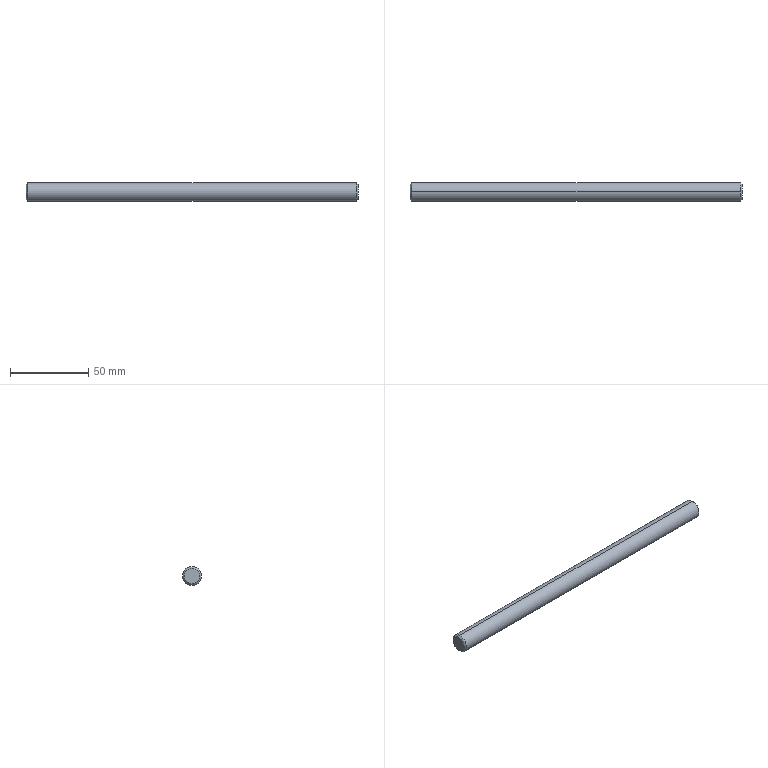Component | SolidWorks | PhotoelectricSlideRod-1 | 1 solid | 8 faces | box 212 x 12 x 12 mm | volume 23941 mm3 | cone 4 | cylinder 2 | plane 2 | commonest cylinder face diameters 12 x2
build123d program:
from build123d import *


with BuildPart() as part:
    # Sketch1 → Revolve1 (revolve)
    with BuildSketch(Plane(origin=(0, 0, 0), x_dir=(1, 0, 0), z_dir=(0, 1, 0))):
        Polygon((5, 106), (0, 106), (0, -106), (5, -106), (6, -105), (6, 105), align=None)
    revolve(axis=Axis((0, 0, -106), (0, 0, 1)))


solid = part.part

# Placed as in the assembly
solid = solid.moved(Location((170, 556, -227.5), (0, 90, 0)))
STEP:
#1=COLOUR_RGB('',0.7922,0.8196,0.9333);
#2=FILL_AREA_STYLE_COLOUR('',#1);
#3=FILL_AREA_STYLE('',(#2));
#4=SURFACE_STYLE_FILL_AREA(#3);
#5=SURFACE_SIDE_STYLE('',(#4));
#6=SURFACE_STYLE_USAGE(.BOTH.,#5);
#7=PRESENTATION_STYLE_ASSIGNMENT((#6));
#8=CARTESIAN_POINT('',(10.866,21.89,-9.154));
#9=VERTEX_POINT('',#8);
#10=CARTESIAN_POINT('',(10.866,21.89,-8.76));
#11=VERTEX_POINT('',#10);
#12=CARTESIAN_POINT('',(10.866,21.89,-8.957));
#13=DIRECTION('',(1.,0.,0.));
#14=DIRECTION('',(0.,0.,-1.));
#15=AXIS2_PLACEMENT_3D('',#12,#13,#14);
#16=CIRCLE('',#15,0.1969);
#17=EDGE_CURVE('',#9,#11,#16,.T.);
#18=ORIENTED_EDGE('',*,*,#17,.F.);
#19=CARTESIAN_POINT('',(10.827,21.89,-9.193));
#20=VERTEX_POINT('',#19);
#21=CARTESIAN_POINT('',(10.866,21.89,-9.154));
#22=DIRECTION('',(-0.7071,-0.,-0.7071));
#23=VECTOR('',#22,39.37);
#24=LINE('',#21,#23);
#25=EDGE_CURVE('',#9,#20,#24,.T.);
#26=ORIENTED_EDGE('',*,*,#25,.T.);
#27=CARTESIAN_POINT('',(10.827,21.89,-8.72));
#28=VERTEX_POINT('',#27);
#29=CARTESIAN_POINT('',(10.827,21.89,-8.957));
#30=DIRECTION('',(1.,0.,0.));
#31=DIRECTION('',(0.,0.,-1.));
#32=AXIS2_PLACEMENT_3D('',#29,#30,#31);
#33=CIRCLE('',#32,0.2362);
#34=EDGE_CURVE('',#20,#28,#33,.T.);
#35=ORIENTED_EDGE('',*,*,#34,.T.);
#36=CARTESIAN_POINT('',(10.866,21.89,-8.76));
#37=DIRECTION('',(-0.7071,-0.,0.7071));
#38=VECTOR('',#37,39.37);
#39=LINE('',#36,#38);
#40=EDGE_CURVE('',#11,#28,#39,.T.);
#41=ORIENTED_EDGE('',*,*,#40,.F.);
#42=EDGE_LOOP('',(#18,#26,#35,#41));
#43=FACE_OUTER_BOUND('',#42,.T.);
#44=CARTESIAN_POINT('',(10.866,21.89,-8.957));
#45=DIRECTION('',(-1.,-0.,0.));
#46=DIRECTION('',(0.,0.,1.));
#47=AXIS2_PLACEMENT_3D('',#44,#45,#46);
#48=CONICAL_SURFACE('',#47,0.1969,0.7854);
#49=ADVANCED_FACE('',(#43),#48,.T.);
#50=CARTESIAN_POINT('',(2.559,21.89,-9.193));
#51=VERTEX_POINT('',#50);
#52=CARTESIAN_POINT('',(2.559,21.89,-8.72));
#53=VERTEX_POINT('',#52);
#54=CARTESIAN_POINT('',(2.559,21.89,-8.957));
#55=DIRECTION('',(1.,0.,0.));
#56=DIRECTION('',(0.,0.,-1.));
#57=AXIS2_PLACEMENT_3D('',#54,#55,#56);
#58=CIRCLE('',#57,0.2362);
#59=EDGE_CURVE('',#51,#53,#58,.T.);
#60=ORIENTED_EDGE('',*,*,#59,.T.);
#61=CARTESIAN_POINT('',(2.52,21.89,-8.72));
#62=DIRECTION('',(1.,0.,0.));
#63=VECTOR('',#62,39.37);
#64=LINE('',#61,#63);
#65=EDGE_CURVE('',#53,#28,#64,.T.);
#66=ORIENTED_EDGE('',*,*,#65,.T.);
#67=ORIENTED_EDGE('',*,*,#34,.F.);
#68=CARTESIAN_POINT('',(2.52,21.89,-9.193));
#69=DIRECTION('',(1.,0.,0.));
#70=VECTOR('',#69,39.37);
#71=LINE('',#68,#70);
#72=EDGE_CURVE('',#51,#20,#71,.T.);
#73=ORIENTED_EDGE('',*,*,#72,.F.);
#74=EDGE_LOOP('',(#60,#66,#67,#73));
#75=FACE_OUTER_BOUND('',#74,.T.);
#76=CARTESIAN_POINT('',(2.52,21.89,-8.957));
#77=DIRECTION('',(1.,0.,0.));
#78=DIRECTION('',(0.,0.,-1.));
#79=AXIS2_PLACEMENT_3D('',#76,#77,#78);
#80=CYLINDRICAL_SURFACE('',#79,0.2362);
#81=ADVANCED_FACE('',(#75),#80,.T.);
#82=CARTESIAN_POINT('',(2.52,21.89,-9.154));
#83=VERTEX_POINT('',#82);
#84=CARTESIAN_POINT('',(2.52,21.89,-8.76));
#85=VERTEX_POINT('',#84);
#86=CARTESIAN_POINT('',(2.52,21.89,-8.957));
#87=DIRECTION('',(1.,0.,0.));
#88=DIRECTION('',(0.,0.,-1.));
#89=AXIS2_PLACEMENT_3D('',#86,#87,#88);
#90=CIRCLE('',#89,0.1969);
#91=EDGE_CURVE('',#83,#85,#90,.T.);
#92=ORIENTED_EDGE('',*,*,#91,.T.);
#93=CARTESIAN_POINT('',(2.559,21.89,-8.72));
#94=DIRECTION('',(0.7071,0.,0.7071));
#95=VECTOR('',#94,39.37);
#96=LINE('',#93,#95);
#97=EDGE_CURVE('',#85,#53,#96,.T.);
#98=ORIENTED_EDGE('',*,*,#97,.T.);
#99=ORIENTED_EDGE('',*,*,#59,.F.);
#100=CARTESIAN_POINT('',(2.559,21.89,-9.193));
#101=DIRECTION('',(0.7071,-0.,-0.7071));
#102=VECTOR('',#101,39.37);
#103=LINE('',#100,#102);
#104=EDGE_CURVE('',#83,#51,#103,.T.);
#105=ORIENTED_EDGE('',*,*,#104,.F.);
#106=EDGE_LOOP('',(#92,#98,#99,#105));
#107=FACE_OUTER_BOUND('',#106,.T.);
#108=CARTESIAN_POINT('',(2.559,21.89,-8.957));
#109=DIRECTION('',(1.,0.,0.));
#110=DIRECTION('',(0.,0.,-1.));
#111=AXIS2_PLACEMENT_3D('',#108,#109,#110);
#112=CONICAL_SURFACE('',#111,0.2362,0.7854);
#113=ADVANCED_FACE('',(#107),#112,.T.);
#114=ORIENTED_EDGE('',*,*,#97,.F.);
#115=CARTESIAN_POINT('',(2.52,21.89,-8.957));
#116=DIRECTION('',(1.,0.,0.));
#117=DIRECTION('',(0.,0.,-1.));
#118=AXIS2_PLACEMENT_3D('',#115,#116,#117);
#119=CIRCLE('',#118,0.1969);
#120=EDGE_CURVE('',#85,#83,#119,.T.);
#121=ORIENTED_EDGE('',*,*,#120,.T.);
#122=ORIENTED_EDGE('',*,*,#104,.T.);
#123=CARTESIAN_POINT('',(2.559,21.89,-8.957));
#124=DIRECTION('',(1.,0.,0.));
#125=DIRECTION('',(0.,0.,-1.));
#126=AXIS2_PLACEMENT_3D('',#123,#124,#125);
#127=CIRCLE('',#126,0.2362);
#128=EDGE_CURVE('',#53,#51,#127,.T.);
#129=ORIENTED_EDGE('',*,*,#128,.F.);
#130=EDGE_LOOP('',(#114,#121,#122,#129));
#131=FACE_OUTER_BOUND('',#130,.T.);
#132=CARTESIAN_POINT('',(2.559,21.89,-8.957));
#133=DIRECTION('',(1.,0.,0.));
#134=DIRECTION('',(0.,0.,-1.));
#135=AXIS2_PLACEMENT_3D('',#132,#133,#134);
#136=CONICAL_SURFACE('',#135,0.2362,0.7854);
#137=ADVANCED_FACE('',(#131),#136,.T.);
#138=ORIENTED_EDGE('',*,*,#65,.F.);
#139=ORIENTED_EDGE('',*,*,#128,.T.);
#140=ORIENTED_EDGE('',*,*,#72,.T.);
#141=CARTESIAN_POINT('',(10.827,21.89,-8.957));
#142=DIRECTION('',(1.,0.,0.));
#143=DIRECTION('',(0.,0.,-1.));
#144=AXIS2_PLACEMENT_3D('',#141,#142,#143);
#145=CIRCLE('',#144,0.2362);
#146=EDGE_CURVE('',#28,#20,#145,.T.);
#147=ORIENTED_EDGE('',*,*,#146,.F.);
#148=EDGE_LOOP('',(#138,#139,#140,#147));
#149=FACE_OUTER_BOUND('',#148,.T.);
#150=CARTESIAN_POINT('',(2.52,21.89,-8.957));
#151=DIRECTION('',(1.,0.,0.));
#152=DIRECTION('',(0.,0.,-1.));
#153=AXIS2_PLACEMENT_3D('',#150,#151,#152);
#154=CYLINDRICAL_SURFACE('',#153,0.2362);
#155=ADVANCED_FACE('',(#149),#154,.T.);
#156=ORIENTED_EDGE('',*,*,#25,.F.);
#157=CARTESIAN_POINT('',(10.866,21.89,-8.957));
#158=DIRECTION('',(1.,0.,0.));
#159=DIRECTION('',(0.,0.,-1.));
#160=AXIS2_PLACEMENT_3D('',#157,#158,#159);
#161=CIRCLE('',#160,0.1969);
#162=EDGE_CURVE('',#11,#9,#161,.T.);
#163=ORIENTED_EDGE('',*,*,#162,.F.);
#164=ORIENTED_EDGE('',*,*,#40,.T.);
#165=ORIENTED_EDGE('',*,*,#146,.T.);
#166=EDGE_LOOP('',(#156,#163,#164,#165));
#167=FACE_OUTER_BOUND('',#166,.T.);
#168=CARTESIAN_POINT('',(10.866,21.89,-8.957));
#169=DIRECTION('',(-1.,-0.,0.));
#170=DIRECTION('',(0.,0.,1.));
#171=AXIS2_PLACEMENT_3D('',#168,#169,#170);
#172=CONICAL_SURFACE('',#171,0.1969,0.7854);
#173=ADVANCED_FACE('',(#167),#172,.T.);
#174=ORIENTED_EDGE('',*,*,#162,.T.);
#175=ORIENTED_EDGE('',*,*,#17,.T.);
#176=EDGE_LOOP('',(#174,#175));
#177=FACE_OUTER_BOUND('',#176,.T.);
#178=CARTESIAN_POINT('',(10.866,21.89,-8.957));
#179=DIRECTION('',(1.,0.,0.));
#180=DIRECTION('',(0.,-0.,-1.));
#181=AXIS2_PLACEMENT_3D('',#178,#179,#180);
#182=PLANE('',#181);
#183=ADVANCED_FACE('',(#177),#182,.T.);
#184=ORIENTED_EDGE('',*,*,#91,.F.);
#185=ORIENTED_EDGE('',*,*,#120,.F.);
#186=EDGE_LOOP('',(#184,#185));
#187=FACE_OUTER_BOUND('',#186,.T.);
#188=CARTESIAN_POINT('',(2.52,21.89,-9.154));
#189=DIRECTION('',(-1.,-0.,0.));
#190=DIRECTION('',(-0.,0.,1.));
#191=AXIS2_PLACEMENT_3D('',#188,#189,#190);
#192=PLANE('',#191);
#193=ADVANCED_FACE('',(#187),#192,.T.);
#194=CLOSED_SHELL('',(#49,#81,#113,#137,#155,#173,#183,#193));
#195=MANIFOLD_SOLID_BREP('',#194);
#196=STYLED_ITEM('',(#7),#195);
#197=(LENGTH_UNIT()NAMED_UNIT(*)SI_UNIT($,.METRE.));
#198=LENGTH_MEASURE_WITH_UNIT(LENGTH_MEASURE(0.0254),#197);
#199=DIMENSIONAL_EXPONENTS(1.,0.,0.,0.,0.,0.,0.);
#200=(CONVERSION_BASED_UNIT('',#198)LENGTH_UNIT()NAMED_UNIT(#199));
#201=UNCERTAINTY_MEASURE_WITH_UNIT(LENGTH_MEASURE(0.00001),#200,'','');
#202=(NAMED_UNIT(*)PLANE_ANGLE_UNIT()SI_UNIT($,.RADIAN.));
#203=(NAMED_UNIT(*)SI_UNIT($,.STERADIAN.)SOLID_ANGLE_UNIT());
#204=(GEOMETRIC_REPRESENTATION_CONTEXT(3)GLOBAL_UNCERTAINTY_ASSIGNED_CONTEXT((#201))GLOBAL_UNIT_ASSIGNED_CONTEXT((#200,#202,#203))REPRESENTATION_CONTEXT('',''));
#205=MECHANICAL_DESIGN_GEOMETRIC_PRESENTATION_REPRESENTATION('',(#196),#204);
#206=PRESENTATION_LAYER_ASSIGNMENT('','',(#196));
#207=CARTESIAN_POINT('',(0.,0.,0.));
#208=DIRECTION('',(0.,0.,1.));
#209=DIRECTION('',(1.,0.,0.));
#210=AXIS2_PLACEMENT_3D('',#207,#208,#209);
#211=(LENGTH_UNIT()NAMED_UNIT(*)SI_UNIT($,.METRE.));
#212=LENGTH_MEASURE_WITH_UNIT(LENGTH_MEASURE(0.0254),#211);
#213=DIMENSIONAL_EXPONENTS(1.,0.,0.,0.,0.,0.,0.);
#214=(CONVERSION_BASED_UNIT('',#212)LENGTH_UNIT()NAMED_UNIT(#213));
#215=UNCERTAINTY_MEASURE_WITH_UNIT(LENGTH_MEASURE(0.00001),#214,'','');
#216=(NAMED_UNIT(*)PLANE_ANGLE_UNIT()SI_UNIT($,.RADIAN.));
#217=(NAMED_UNIT(*)SI_UNIT($,.STERADIAN.)SOLID_ANGLE_UNIT());
#218=(GEOMETRIC_REPRESENTATION_CONTEXT(3)GLOBAL_UNCERTAINTY_ASSIGNED_CONTEXT((#215))GLOBAL_UNIT_ASSIGNED_CONTEXT((#214,#216,#217))REPRESENTATION_CONTEXT('',''));
#219=ADVANCED_BREP_SHAPE_REPRESENTATION('',(#195,#210),#218);